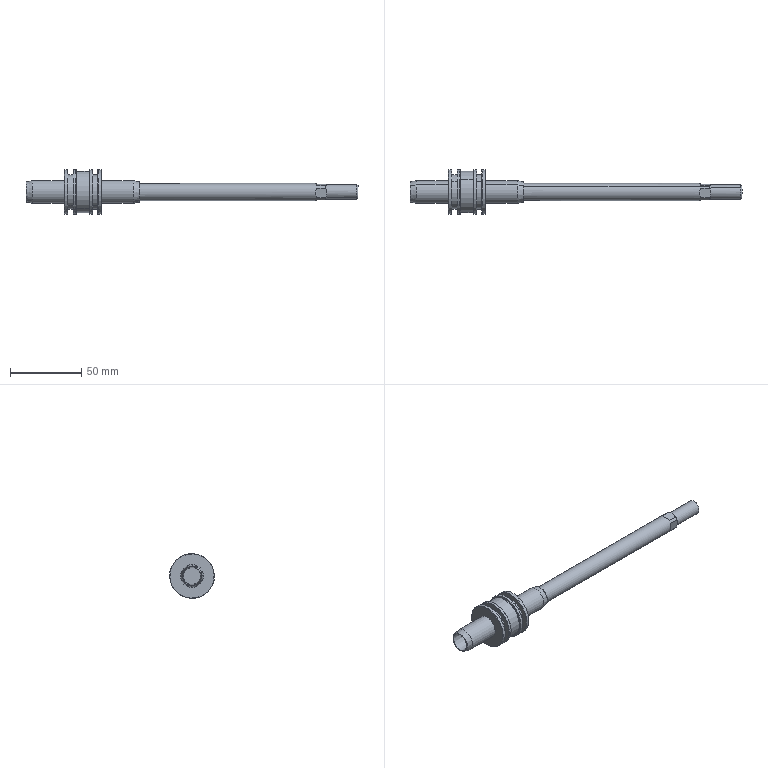Component | SolidWorks | HZ022-SC32x100S-1_HZ022-SC32x100S (2)-1 | 1 solid | 81 faces | volume 38821 mm3 | cone 29 | cylinder 24 | plane 20 | spline 8 | commonest cylinder face diameters 31.5 x8 12 x4 16 x4 24 x4 10 x2 28.92 x2 | material AL6061